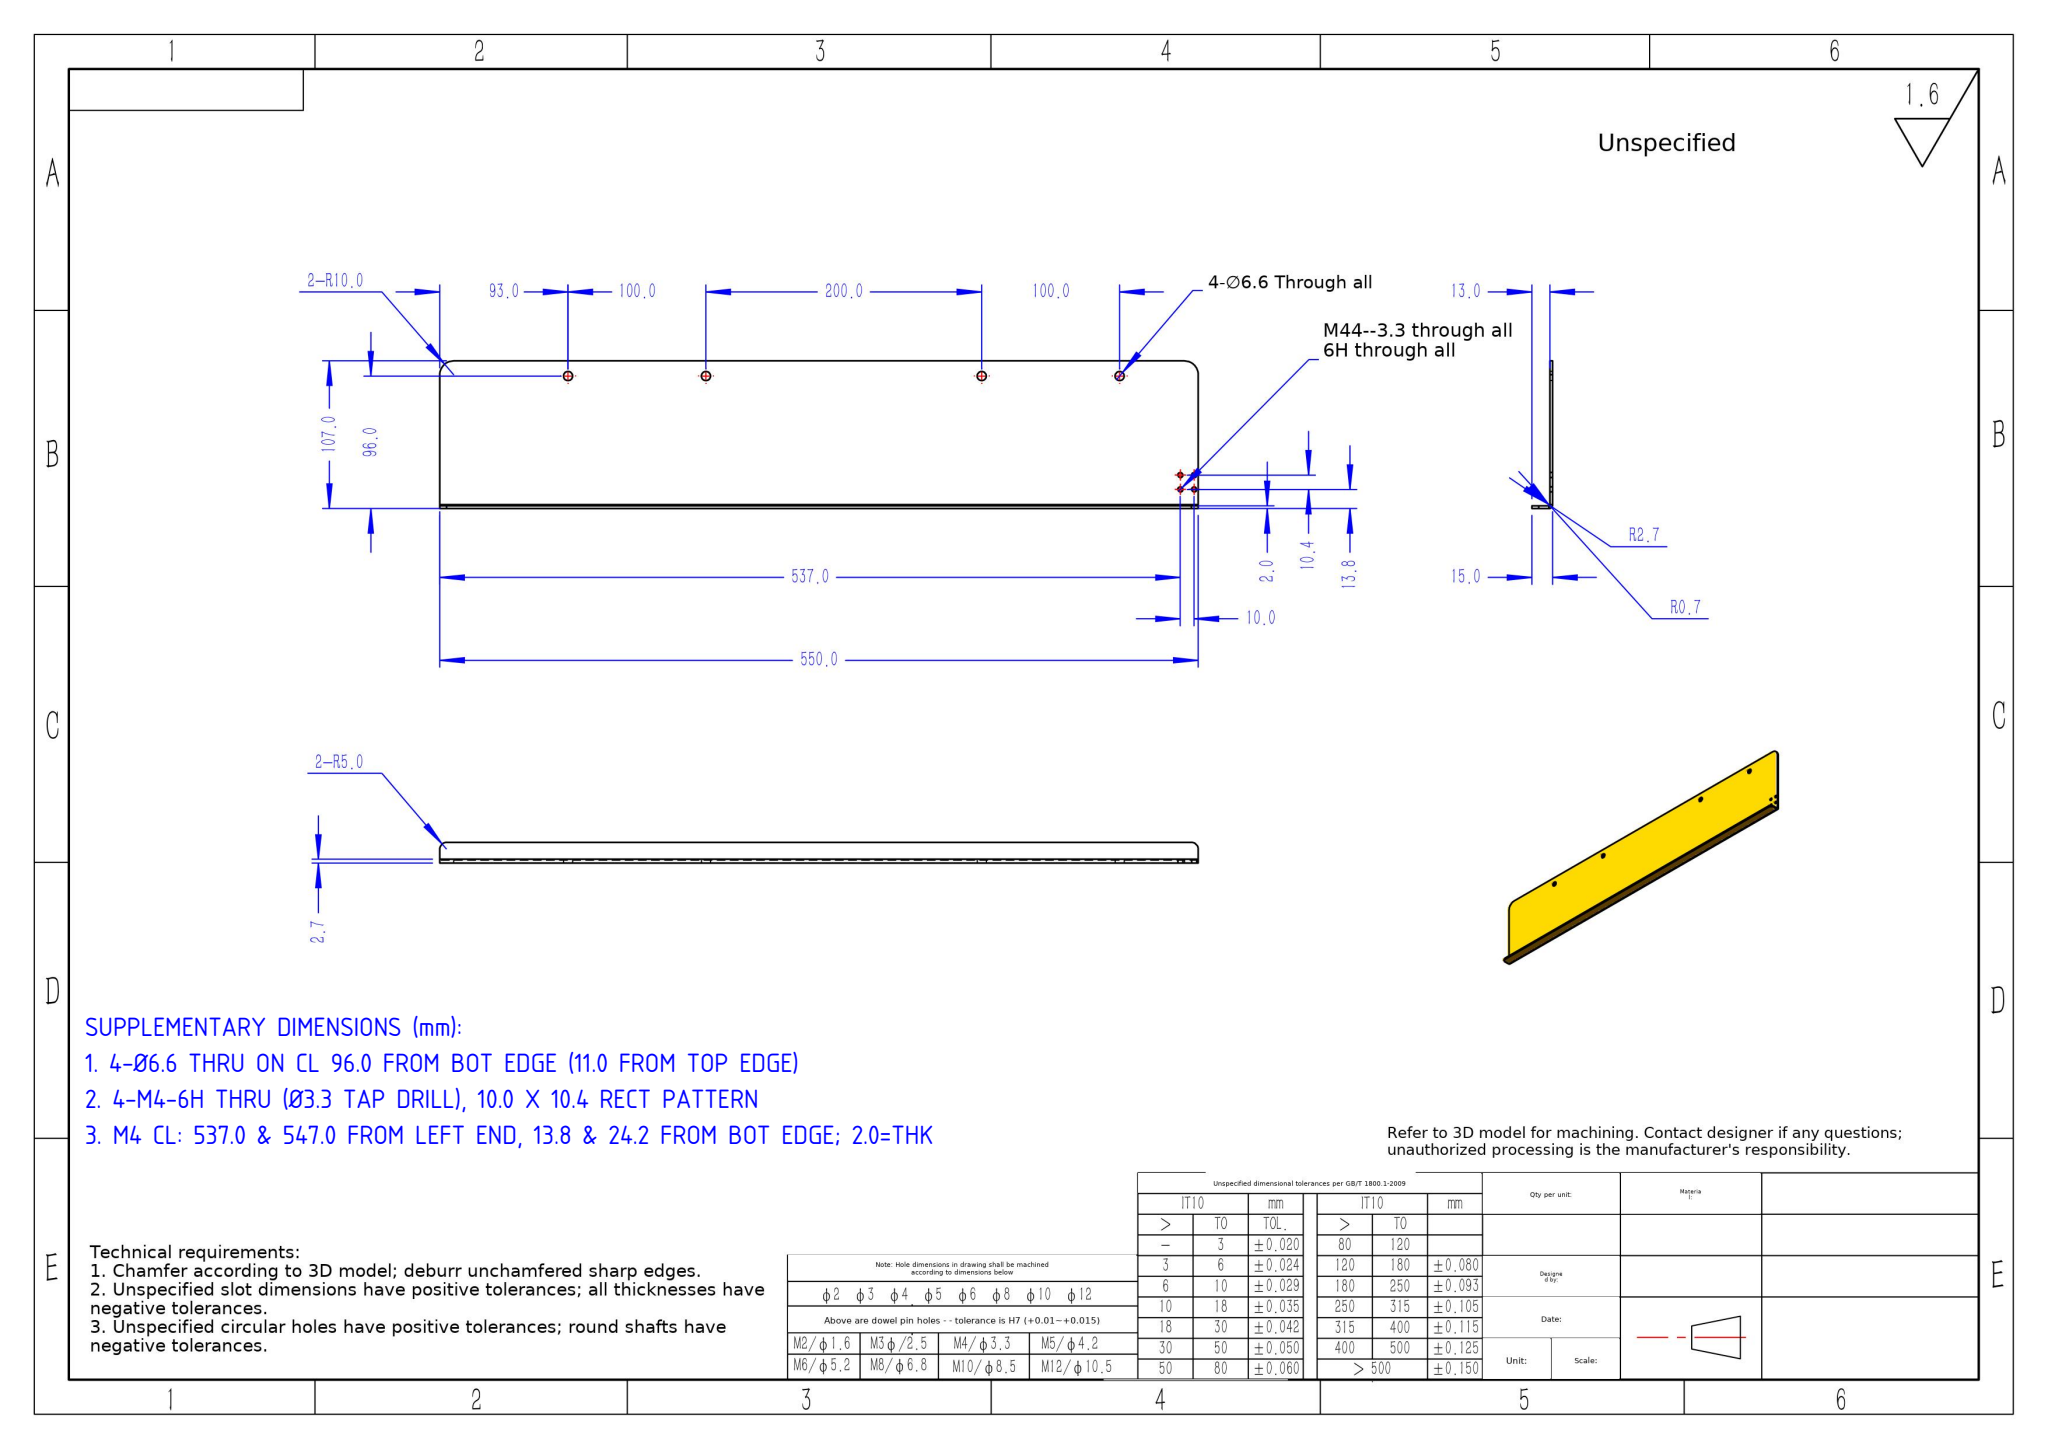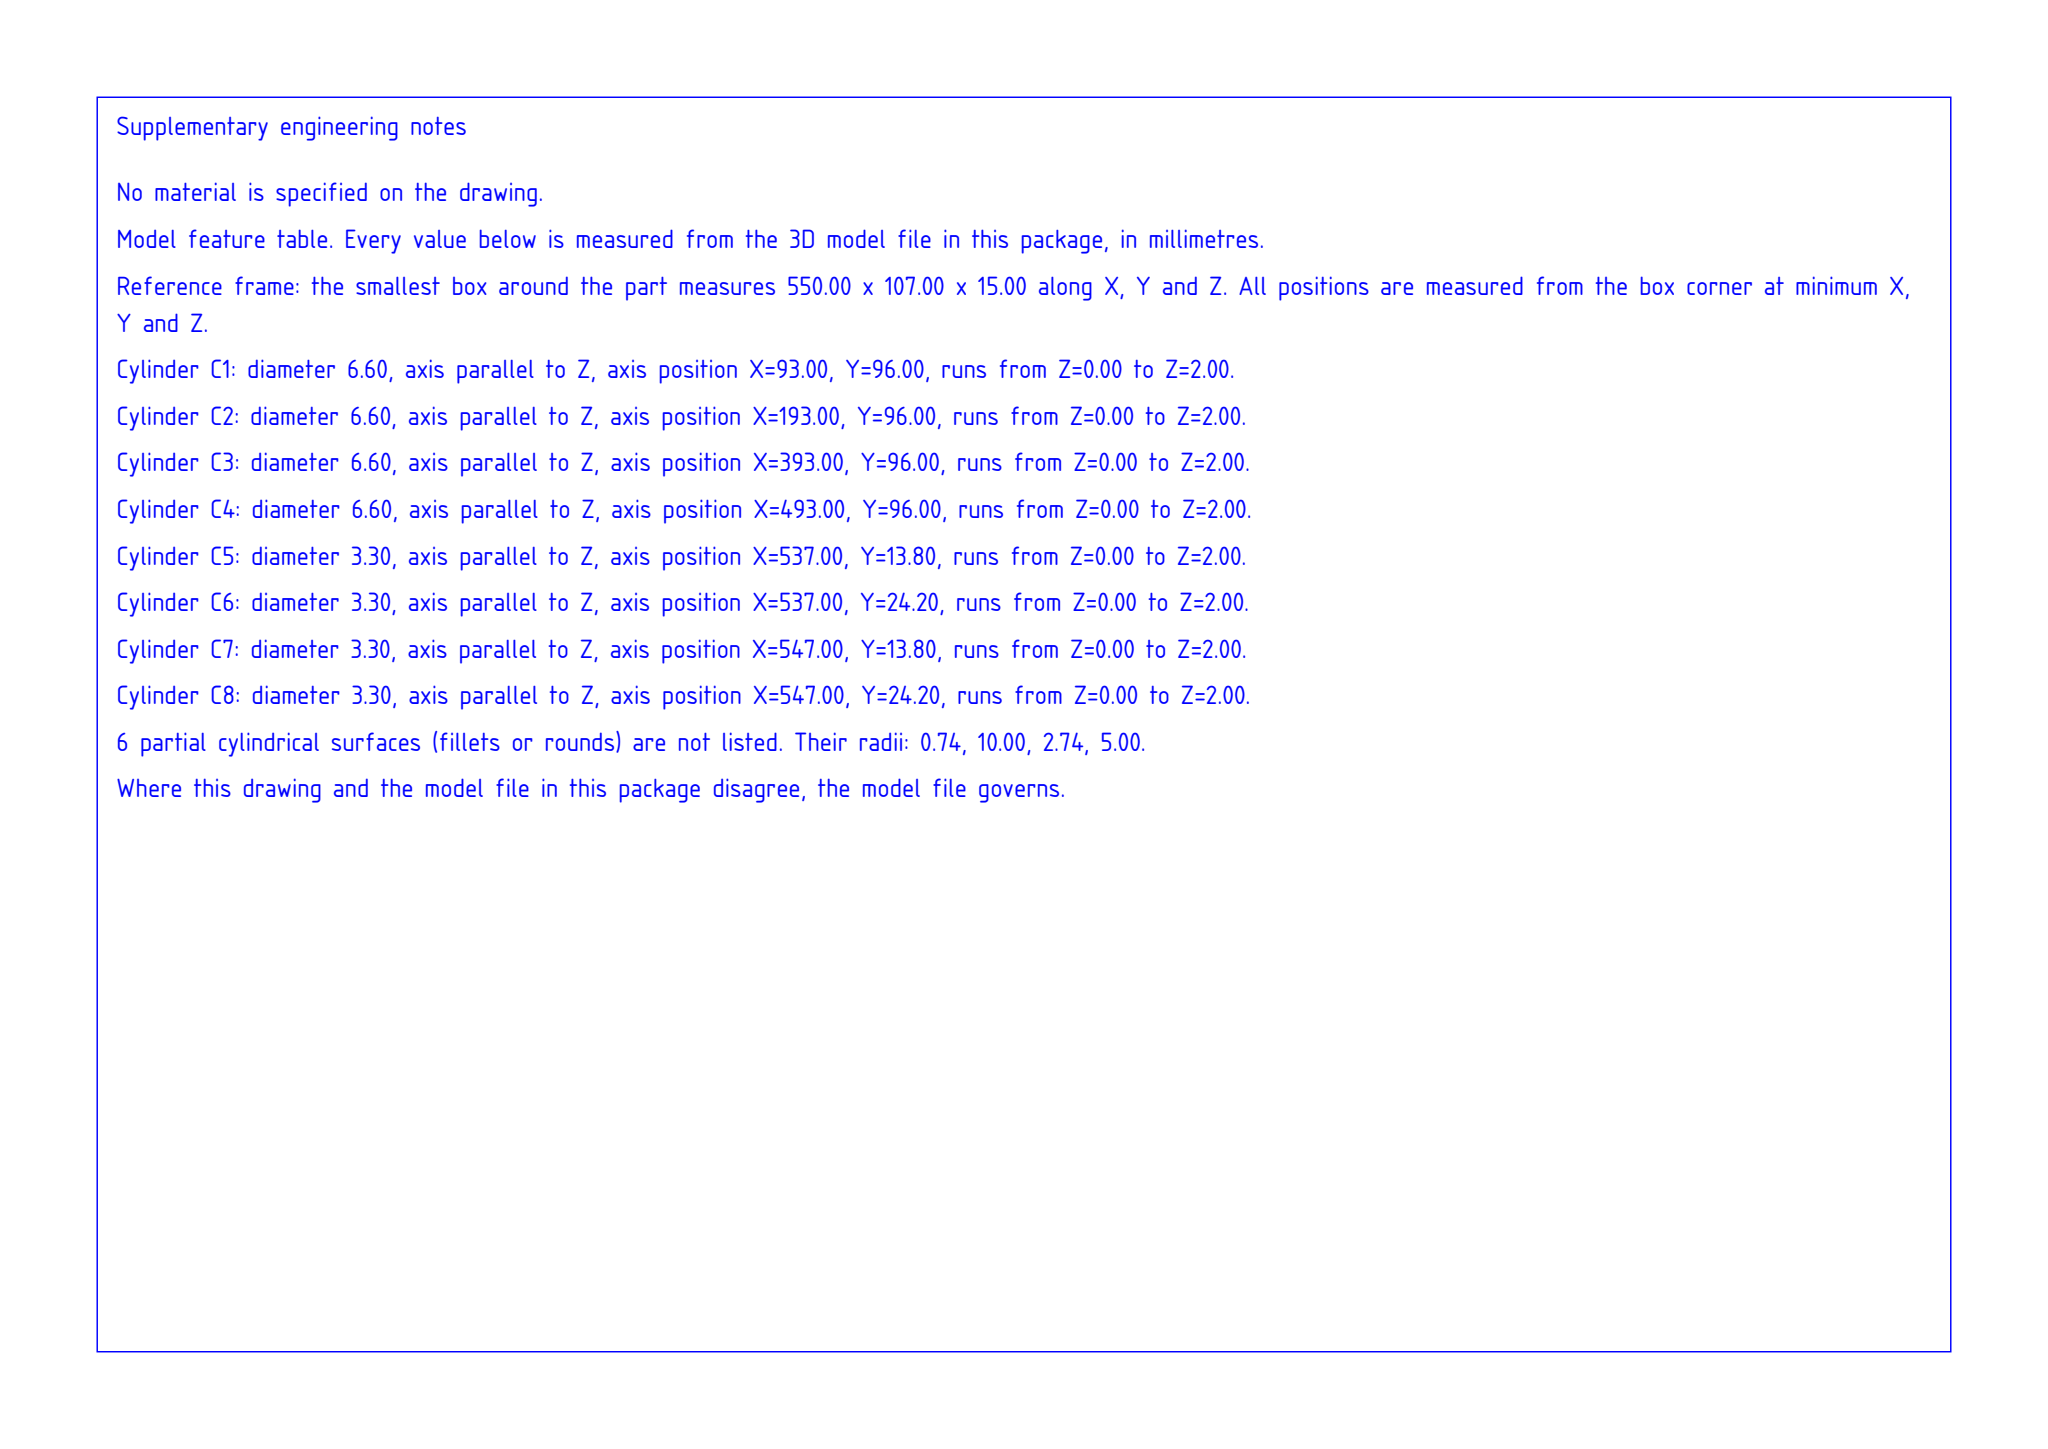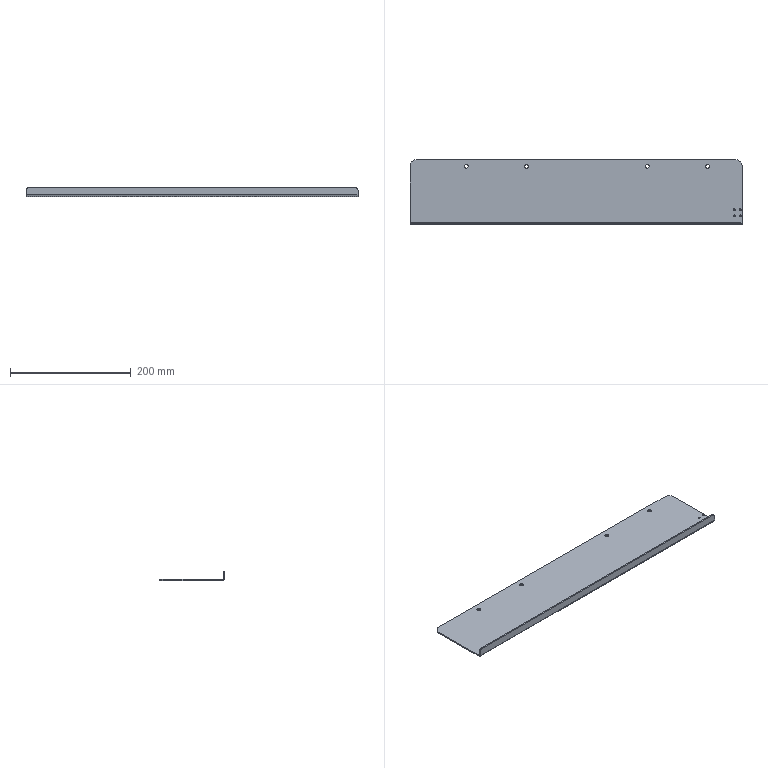Part | SolidWorks | mm | 1 solid | 34 faces | box 550 x 107 x 15 mm | volume 130731 mm3 | cylinder 22 | plane 12 | commonest cylinder face diameters 6.6 x8 3.3 x8 20 x2 10 x2 5.473 x1 1.473 x1